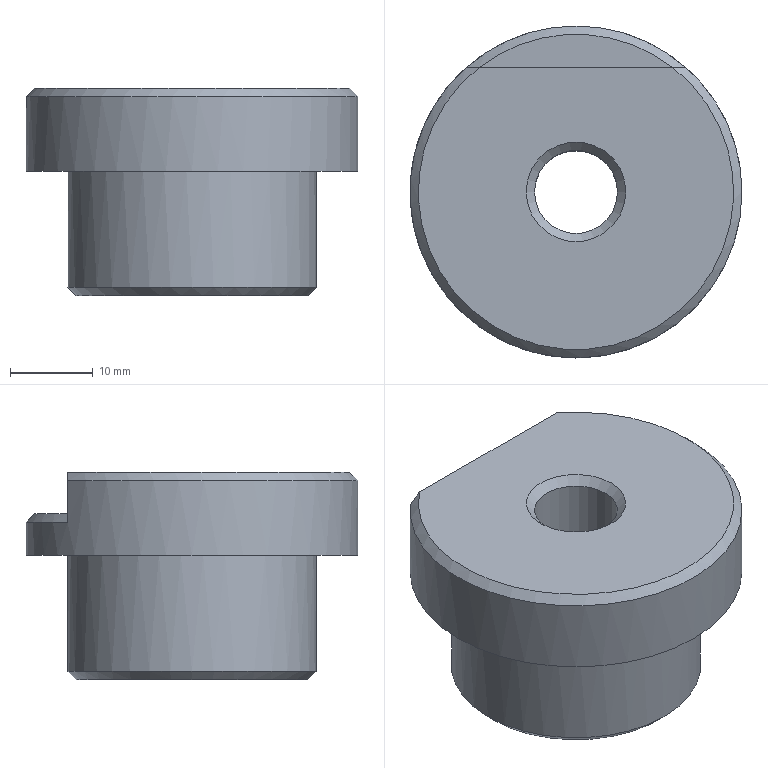Component | NX | DRILL_BUSHING_3 | 1 solid | 12 faces | box 40 x 40 x 25 mm | volume 20628 mm3 | plane 5 | cone 4 | cylinder 3 | commonest cylinder face diameters 40 x1 30 x1 10 x1
STEP:
#1=CARTESIAN_POINT('',(0.,0.,0.));
#2=DIRECTION('',(0.,0.,1.));
#3=DIRECTION('',(1.,0.,0.));
#4=AXIS2_PLACEMENT_3D('',#1,#2,#3);
#5=CARTESIAN_POINT('',(79.34,104.989,375.));
#6=VERTEX_POINT('',#5);
#7=CARTESIAN_POINT('',(59.34,104.989,375.));
#8=DIRECTION('',(0.,0.,1.));
#9=DIRECTION('',(1.,0.,0.));
#10=AXIS2_PLACEMENT_3D('',#7,#8,#9);
#11=CIRCLE('',#10,20.);
#12=CARTESIAN_POINT('',(59.34,104.989,375.));
#13=DIRECTION('',(0.,0.,1.));
#14=DIRECTION('',(1.,0.,0.));
#15=AXIS2_PLACEMENT_3D('',#12,#13,#14);
#16=CYLINDRICAL_SURFACE('',#15,20.);
#17=CARTESIAN_POINT('',(0.,0.));
#18=DIRECTION('',(1.,0.));
#19=VECTOR('',#18,1.);
#20=LINE('',#17,#19);
#21=(GEOMETRIC_REPRESENTATION_CONTEXT(2)PARAMETRIC_REPRESENTATION_CONTEXT()REPRESENTATION_CONTEXT('',''));
#22=DEFINITIONAL_REPRESENTATION('',(#20),#21);
#23=PCURVE('',#16,#22);
#24=CARTESIAN_POINT('',(59.34,104.989,375.));
#25=DIRECTION('',(0.,0.,1.));
#26=DIRECTION('',(1.,0.,0.));
#27=AXIS2_PLACEMENT_3D('',#24,#25,#26);
#28=PLANE('',#27);
#29=CARTESIAN_POINT('',(0.,0.));
#30=DIRECTION('',(1.,0.));
#31=AXIS2_PLACEMENT_2D('',#29,#30);
#32=CIRCLE('',#31,20.);
#33=(GEOMETRIC_REPRESENTATION_CONTEXT(2)PARAMETRIC_REPRESENTATION_CONTEXT()REPRESENTATION_CONTEXT('',''));
#34=DEFINITIONAL_REPRESENTATION('',(#32),#33);
#35=PCURVE('',#28,#34);
#36=SURFACE_CURVE('',#11,(#23,#35),.PCURVE_S1.);
#37=EDGE_CURVE('',#6,#6,#36,.T.);
#38=ORIENTED_EDGE('',*,*,#37,.T.);
#39=CARTESIAN_POINT('',(79.34,104.989,384.));
#40=VERTEX_POINT('',#39);
#41=CARTESIAN_POINT('',(79.34,104.989,375.));
#42=CARTESIAN_POINT('',(79.34,104.989,384.));
#43=B_SPLINE_CURVE_WITH_KNOTS('',1,(#41,#42),.UNSPECIFIED.,.F.,.F.,(2,2),(0.,9.),.PIECEWISE_BEZIER_KNOTS.);
#44=CARTESIAN_POINT('',(6.283,0.));
#45=DIRECTION('',(0.,1.));
#46=VECTOR('',#45,1.);
#47=LINE('',#44,#46);
#48=(GEOMETRIC_REPRESENTATION_CONTEXT(2)PARAMETRIC_REPRESENTATION_CONTEXT()REPRESENTATION_CONTEXT('',''));
#49=DEFINITIONAL_REPRESENTATION('',(#47),#48);
#50=PCURVE('',#16,#49);
#51=CARTESIAN_POINT('',(0.,0.));
#52=DIRECTION('',(0.,1.));
#53=VECTOR('',#52,1.);
#54=LINE('',#51,#53);
#55=(GEOMETRIC_REPRESENTATION_CONTEXT(2)PARAMETRIC_REPRESENTATION_CONTEXT()REPRESENTATION_CONTEXT('',''));
#56=DEFINITIONAL_REPRESENTATION('',(#54),#55);
#57=PCURVE('',#16,#56);
#58=SEAM_CURVE('',#43,(#50,#57),.PCURVE_S1.);
#59=EDGE_CURVE('',#6,#40,#58,.T.);
#60=ORIENTED_EDGE('',*,*,#59,.T.);
#61=CARTESIAN_POINT('',(46.111,119.989,384.));
#62=VERTEX_POINT('',#61);
#63=CARTESIAN_POINT('',(59.34,104.989,384.));
#64=DIRECTION('',(0.,0.,-1.));
#65=DIRECTION('',(1.,0.,0.));
#66=AXIS2_PLACEMENT_3D('',#63,#64,#65);
#67=CIRCLE('',#66,20.);
#68=CARTESIAN_POINT('',(12.566,9.));
#69=DIRECTION('',(-1.,0.));
#70=VECTOR('',#69,1.);
#71=LINE('',#68,#70);
#72=(GEOMETRIC_REPRESENTATION_CONTEXT(2)PARAMETRIC_REPRESENTATION_CONTEXT()REPRESENTATION_CONTEXT('',''));
#73=DEFINITIONAL_REPRESENTATION('',(#71),#72);
#74=PCURVE('',#16,#73);
#75=CARTESIAN_POINT('',(59.34,104.989,385.));
#76=DIRECTION('',(0.,0.,-1.));
#77=DIRECTION('',(-1.,0.,0.));
#78=AXIS2_PLACEMENT_3D('',#75,#76,#77);
#79=CONICAL_SURFACE('',#78,19.,0.7854);
#80=CARTESIAN_POINT('',(-3.142,1.));
#81=DIRECTION('',(1.,-0.));
#82=VECTOR('',#81,1.);
#83=LINE('',#80,#82);
#84=(GEOMETRIC_REPRESENTATION_CONTEXT(2)PARAMETRIC_REPRESENTATION_CONTEXT()REPRESENTATION_CONTEXT('',''));
#85=DEFINITIONAL_REPRESENTATION('',(#83),#84);
#86=PCURVE('',#79,#85);
#87=SURFACE_CURVE('',#67,(#74,#86),.PCURVE_S1.);
#88=EDGE_CURVE('',#40,#62,#87,.T.);
#89=ORIENTED_EDGE('',*,*,#88,.T.);
#90=CARTESIAN_POINT('',(46.111,119.989,379.));
#91=VERTEX_POINT('',#90);
#92=CARTESIAN_POINT('',(46.111,119.989,375.));
#93=DIRECTION('',(0.,0.,-1.));
#94=VECTOR('',#93,1.);
#95=LINE('',#92,#94);
#96=CARTESIAN_POINT('',(2.294,0.));
#97=DIRECTION('',(0.,-1.));
#98=VECTOR('',#97,1.);
#99=LINE('',#96,#98);
#100=(GEOMETRIC_REPRESENTATION_CONTEXT(2)PARAMETRIC_REPRESENTATION_CONTEXT()REPRESENTATION_CONTEXT('',''));
#101=DEFINITIONAL_REPRESENTATION('',(#99),#100);
#102=PCURVE('',#16,#101);
#103=CARTESIAN_POINT('',(159.34,119.989,394.));
#104=DIRECTION('',(0.,1.,0.));
#105=DIRECTION('',(0.,-0.,1.));
#106=AXIS2_PLACEMENT_3D('',#103,#104,#105);
#107=PLANE('',#106);
#108=CARTESIAN_POINT('',(-19.,-113.229));
#109=DIRECTION('',(-1.,0.));
#110=VECTOR('',#109,1.);
#111=LINE('',#108,#110);
#112=(GEOMETRIC_REPRESENTATION_CONTEXT(2)PARAMETRIC_REPRESENTATION_CONTEXT()REPRESENTATION_CONTEXT('',''));
#113=DEFINITIONAL_REPRESENTATION('',(#111),#112);
#114=PCURVE('',#107,#113);
#115=SURFACE_CURVE('',#95,(#102,#114),.PCURVE_S1.);
#116=EDGE_CURVE('',#62,#91,#115,.T.);
#117=ORIENTED_EDGE('',*,*,#116,.T.);
#118=CARTESIAN_POINT('',(72.569,119.989,379.));
#119=VERTEX_POINT('',#118);
#120=CARTESIAN_POINT('',(59.34,104.989,379.));
#121=DIRECTION('',(0.,0.,-1.));
#122=DIRECTION('',(1.,0.,0.));
#123=AXIS2_PLACEMENT_3D('',#120,#121,#122);
#124=CIRCLE('',#123,20.);
#125=CARTESIAN_POINT('',(6.283,4.));
#126=DIRECTION('',(-1.,0.));
#127=VECTOR('',#126,1.);
#128=LINE('',#125,#127);
#129=(GEOMETRIC_REPRESENTATION_CONTEXT(2)PARAMETRIC_REPRESENTATION_CONTEXT()REPRESENTATION_CONTEXT('',''));
#130=DEFINITIONAL_REPRESENTATION('',(#128),#129);
#131=PCURVE('',#16,#130);
#132=CARTESIAN_POINT('',(59.34,104.989,379.));
#133=DIRECTION('',(0.,0.,-1.));
#134=DIRECTION('',(-1.,0.,0.));
#135=AXIS2_PLACEMENT_3D('',#132,#133,#134);
#136=CONICAL_SURFACE('',#135,20.,0.7854);
#137=CARTESIAN_POINT('',(-3.142,0.));
#138=DIRECTION('',(1.,0.));
#139=VECTOR('',#138,1.);
#140=LINE('',#137,#139);
#141=(GEOMETRIC_REPRESENTATION_CONTEXT(2)PARAMETRIC_REPRESENTATION_CONTEXT()REPRESENTATION_CONTEXT('',''));
#142=DEFINITIONAL_REPRESENTATION('',(#140),#141);
#143=PCURVE('',#136,#142);
#144=SURFACE_CURVE('',#124,(#131,#143),.PCURVE_S1.);
#145=EDGE_CURVE('',#91,#119,#144,.T.);
#146=ORIENTED_EDGE('',*,*,#145,.T.);
#147=CARTESIAN_POINT('',(72.569,119.989,384.));
#148=VERTEX_POINT('',#147);
#149=CARTESIAN_POINT('',(72.569,119.989,375.));
#150=DIRECTION('',(0.,0.,1.));
#151=VECTOR('',#150,1.);
#152=LINE('',#149,#151);
#153=CARTESIAN_POINT('',(0.8481,0.));
#154=DIRECTION('',(0.,1.));
#155=VECTOR('',#154,1.);
#156=LINE('',#153,#155);
#157=(GEOMETRIC_REPRESENTATION_CONTEXT(2)PARAMETRIC_REPRESENTATION_CONTEXT()REPRESENTATION_CONTEXT('',''));
#158=DEFINITIONAL_REPRESENTATION('',(#156),#157);
#159=PCURVE('',#16,#158);
#160=CARTESIAN_POINT('',(-19.,-86.771));
#161=DIRECTION('',(1.,0.));
#162=VECTOR('',#161,1.);
#163=LINE('',#160,#162);
#164=(GEOMETRIC_REPRESENTATION_CONTEXT(2)PARAMETRIC_REPRESENTATION_CONTEXT()REPRESENTATION_CONTEXT('',''));
#165=DEFINITIONAL_REPRESENTATION('',(#163),#164);
#166=PCURVE('',#107,#165);
#167=SURFACE_CURVE('',#152,(#159,#166),.PCURVE_S1.);
#168=EDGE_CURVE('',#119,#148,#167,.T.);
#169=ORIENTED_EDGE('',*,*,#168,.T.);
#170=CARTESIAN_POINT('',(59.34,104.989,384.));
#171=DIRECTION('',(0.,0.,-1.));
#172=DIRECTION('',(1.,0.,0.));
#173=AXIS2_PLACEMENT_3D('',#170,#171,#172);
#174=CIRCLE('',#173,20.);
#175=CARTESIAN_POINT('',(6.283,9.));
#176=DIRECTION('',(-1.,0.));
#177=VECTOR('',#176,1.);
#178=LINE('',#175,#177);
#179=(GEOMETRIC_REPRESENTATION_CONTEXT(2)PARAMETRIC_REPRESENTATION_CONTEXT()REPRESENTATION_CONTEXT('',''));
#180=DEFINITIONAL_REPRESENTATION('',(#178),#179);
#181=PCURVE('',#16,#180);
#182=CARTESIAN_POINT('',(-3.142,1.));
#183=DIRECTION('',(1.,0.));
#184=VECTOR('',#183,1.);
#185=LINE('',#182,#184);
#186=(GEOMETRIC_REPRESENTATION_CONTEXT(2)PARAMETRIC_REPRESENTATION_CONTEXT()REPRESENTATION_CONTEXT('',''));
#187=DEFINITIONAL_REPRESENTATION('',(#185),#186);
#188=PCURVE('',#79,#187);
#189=SURFACE_CURVE('',#174,(#181,#188),.PCURVE_S1.);
#190=EDGE_CURVE('',#148,#40,#189,.T.);
#191=ORIENTED_EDGE('',*,*,#190,.T.);
#192=ORIENTED_EDGE('',*,*,#59,.F.);
#193=EDGE_LOOP('',(#38,#60,#89,#117,#146,#169,#191,#192));
#194=FACE_BOUND('',#193,.T.);
#195=ADVANCED_FACE('',(#194),#16,.T.);
#196=CARTESIAN_POINT('',(65.34,104.989,385.));
#197=VERTEX_POINT('',#196);
#198=CARTESIAN_POINT('',(59.34,104.989,385.));
#199=DIRECTION('',(0.,0.,-1.));
#200=DIRECTION('',(1.,0.,0.));
#201=AXIS2_PLACEMENT_3D('',#198,#199,#200);
#202=CIRCLE('',#201,6.);
#203=CARTESIAN_POINT('',(59.34,104.989,385.));
#204=DIRECTION('',(0.,0.,1.));
#205=DIRECTION('',(1.,0.,0.));
#206=AXIS2_PLACEMENT_3D('',#203,#204,#205);
#207=PLANE('',#206);
#208=CARTESIAN_POINT('',(6.,0.));
#209=CARTESIAN_POINT('',(6.,-10.392));
#210=CARTESIAN_POINT('',(-3.,-5.196));
#211=CARTESIAN_POINT('',(-12.,-0.));
#212=CARTESIAN_POINT('',(-3.,5.196));
#213=CARTESIAN_POINT('',(6.,10.392));
#214=CARTESIAN_POINT('',(6.,0.));
#215=(BOUNDED_CURVE()B_SPLINE_CURVE(2,(#208,#209,#210,#211,#212,#213,#214),.UNSPECIFIED.,.T.,.F.)B_SPLINE_CURVE_WITH_KNOTS((1,2,2,2,2,1),(-2.094,0.,2.094,4.189,6.283,8.378),.UNSPECIFIED.)CURVE()GEOMETRIC_REPRESENTATION_ITEM()RATIONAL_B_SPLINE_CURVE((1.,0.5,1.,0.5,1.,0.5,1.))REPRESENTATION_ITEM(''));
#216=(GEOMETRIC_REPRESENTATION_CONTEXT(2)PARAMETRIC_REPRESENTATION_CONTEXT()REPRESENTATION_CONTEXT('',''));
#217=DEFINITIONAL_REPRESENTATION('',(#215),#216);
#218=PCURVE('',#207,#217);
#219=CARTESIAN_POINT('',(59.34,104.989,384.));
#220=DIRECTION('',(0.,0.,1.));
#221=DIRECTION('',(1.,0.,0.));
#222=AXIS2_PLACEMENT_3D('',#219,#220,#221);
#223=CONICAL_SURFACE('',#222,5.,0.7854);
#224=CARTESIAN_POINT('',(6.283,1.));
#225=DIRECTION('',(-1.,0.));
#226=VECTOR('',#225,1.);
#227=LINE('',#224,#226);
#228=(GEOMETRIC_REPRESENTATION_CONTEXT(2)PARAMETRIC_REPRESENTATION_CONTEXT()REPRESENTATION_CONTEXT('',''));
#229=DEFINITIONAL_REPRESENTATION('',(#227),#228);
#230=PCURVE('',#223,#229);
#231=SURFACE_CURVE('',#202,(#218,#230),.PCURVE_S1.);
#232=EDGE_CURVE('',#197,#197,#231,.T.);
#233=ORIENTED_EDGE('',*,*,#232,.T.);
#234=EDGE_LOOP('',(#233));
#235=FACE_BOUND('',#234,.T.);
#236=CARTESIAN_POINT('',(71.002,119.989,385.));
#237=VERTEX_POINT('',#236);
#238=CARTESIAN_POINT('',(47.678,119.989,385.));
#239=VERTEX_POINT('',#238);
#240=CARTESIAN_POINT('',(59.34,119.989,385.));
#241=DIRECTION('',(-1.,0.,0.));
#242=VECTOR('',#241,1.);
#243=LINE('',#240,#242);
#244=CARTESIAN_POINT('',(0.,15.));
#245=DIRECTION('',(-1.,0.));
#246=VECTOR('',#245,1.);
#247=LINE('',#244,#246);
#248=(GEOMETRIC_REPRESENTATION_CONTEXT(2)PARAMETRIC_REPRESENTATION_CONTEXT()REPRESENTATION_CONTEXT('',''));
#249=DEFINITIONAL_REPRESENTATION('',(#247),#248);
#250=PCURVE('',#207,#249);
#251=CARTESIAN_POINT('',(-9.,-100.));
#252=DIRECTION('',(0.,-1.));
#253=VECTOR('',#252,1.);
#254=LINE('',#251,#253);
#255=(GEOMETRIC_REPRESENTATION_CONTEXT(2)PARAMETRIC_REPRESENTATION_CONTEXT()REPRESENTATION_CONTEXT('',''));
#256=DEFINITIONAL_REPRESENTATION('',(#254),#255);
#257=PCURVE('',#107,#256);
#258=SURFACE_CURVE('',#243,(#250,#257),.PCURVE_S1.);
#259=EDGE_CURVE('',#237,#239,#258,.T.);
#260=ORIENTED_EDGE('',*,*,#259,.T.);
#261=CARTESIAN_POINT('',(59.34,104.989,385.));
#262=DIRECTION('',(0.,0.,1.));
#263=DIRECTION('',(1.,0.,0.));
#264=AXIS2_PLACEMENT_3D('',#261,#262,#263);
#265=CIRCLE('',#264,19.);
#266=CARTESIAN_POINT('',(0.,0.));
#267=DIRECTION('',(1.,0.));
#268=AXIS2_PLACEMENT_2D('',#266,#267);
#269=CIRCLE('',#268,19.);
#270=(GEOMETRIC_REPRESENTATION_CONTEXT(2)PARAMETRIC_REPRESENTATION_CONTEXT()REPRESENTATION_CONTEXT('',''));
#271=DEFINITIONAL_REPRESENTATION('',(#269),#270);
#272=PCURVE('',#207,#271);
#273=CARTESIAN_POINT('',(9.425,0.));
#274=DIRECTION('',(-1.,-0.));
#275=VECTOR('',#274,1.);
#276=LINE('',#273,#275);
#277=(GEOMETRIC_REPRESENTATION_CONTEXT(2)PARAMETRIC_REPRESENTATION_CONTEXT()REPRESENTATION_CONTEXT('',''));
#278=DEFINITIONAL_REPRESENTATION('',(#276),#277);
#279=PCURVE('',#79,#278);
#280=SURFACE_CURVE('',#265,(#272,#279),.PCURVE_S1.);
#281=EDGE_CURVE('',#239,#237,#280,.T.);
#282=ORIENTED_EDGE('',*,*,#281,.T.);
#283=EDGE_LOOP('',(#260,#282));
#284=FACE_BOUND('',#283,.T.);
#285=ADVANCED_FACE('',(#235,#284),#207,.T.);
#286=CARTESIAN_POINT('',(74.34,104.989,375.));
#287=VERTEX_POINT('',#286);
#288=CARTESIAN_POINT('',(59.34,104.989,375.));
#289=DIRECTION('',(0.,0.,-1.));
#290=DIRECTION('',(1.,0.,0.));
#291=AXIS2_PLACEMENT_3D('',#288,#289,#290);
#292=CIRCLE('',#291,15.);
#293=CARTESIAN_POINT('',(15.,0.));
#294=CARTESIAN_POINT('',(15.,-25.981));
#295=CARTESIAN_POINT('',(-7.5,-12.99));
#296=CARTESIAN_POINT('',(-30.,-0.));
#297=CARTESIAN_POINT('',(-7.5,12.99));
#298=CARTESIAN_POINT('',(15.,25.981));
#299=CARTESIAN_POINT('',(15.,0.));
#300=(BOUNDED_CURVE()B_SPLINE_CURVE(2,(#293,#294,#295,#296,#297,#298,#299),.UNSPECIFIED.,.T.,.F.)B_SPLINE_CURVE_WITH_KNOTS((1,2,2,2,2,1),(-2.094,0.,2.094,4.189,6.283,8.378),.UNSPECIFIED.)CURVE()GEOMETRIC_REPRESENTATION_ITEM()RATIONAL_B_SPLINE_CURVE((1.,0.5,1.,0.5,1.,0.5,1.))REPRESENTATION_ITEM(''));
#301=(GEOMETRIC_REPRESENTATION_CONTEXT(2)PARAMETRIC_REPRESENTATION_CONTEXT()REPRESENTATION_CONTEXT('',''));
#302=DEFINITIONAL_REPRESENTATION('',(#300),#301);
#303=PCURVE('',#28,#302);
#304=CARTESIAN_POINT('',(59.34,104.989,360.));
#305=DIRECTION('',(0.,0.,1.));
#306=DIRECTION('',(1.,0.,0.));
#307=AXIS2_PLACEMENT_3D('',#304,#305,#306);
#308=CYLINDRICAL_SURFACE('',#307,15.);
#309=CARTESIAN_POINT('',(6.283,15.));
#310=DIRECTION('',(-1.,0.));
#311=VECTOR('',#310,1.);
#312=LINE('',#309,#311);
#313=(GEOMETRIC_REPRESENTATION_CONTEXT(2)PARAMETRIC_REPRESENTATION_CONTEXT()REPRESENTATION_CONTEXT('',''));
#314=DEFINITIONAL_REPRESENTATION('',(#312),#313);
#315=PCURVE('',#308,#314);
#316=SURFACE_CURVE('',#292,(#303,#315),.PCURVE_S1.);
#317=EDGE_CURVE('',#287,#287,#316,.T.);
#318=ORIENTED_EDGE('',*,*,#317,.F.);
#319=EDGE_LOOP('',(#318));
#320=FACE_BOUND('',#319,.T.);
#321=ORIENTED_EDGE('',*,*,#37,.F.);
#322=EDGE_LOOP('',(#321));
#323=FACE_BOUND('',#322,.T.);
#324=ADVANCED_FACE('',(#320,#323),#28,.F.);
#325=CARTESIAN_POINT('',(44.34,104.989,361.));
#326=VERTEX_POINT('',#325);
#327=CARTESIAN_POINT('',(74.34,104.989,361.));
#328=VERTEX_POINT('',#327);
#329=CARTESIAN_POINT('',(59.34,104.989,361.));
#330=DIRECTION('',(0.,0.,1.));
#331=DIRECTION('',(-1.,0.,0.));
#332=AXIS2_PLACEMENT_3D('',#329,#330,#331);
#333=CIRCLE('',#332,15.);
#334=CARTESIAN_POINT('',(3.142,1.));
#335=DIRECTION('',(1.,0.));
#336=VECTOR('',#335,1.);
#337=LINE('',#334,#336);
#338=(GEOMETRIC_REPRESENTATION_CONTEXT(2)PARAMETRIC_REPRESENTATION_CONTEXT()REPRESENTATION_CONTEXT('',''));
#339=DEFINITIONAL_REPRESENTATION('',(#337),#338);
#340=PCURVE('',#308,#339);
#341=CARTESIAN_POINT('',(59.34,104.989,360.));
#342=DIRECTION('',(0.,0.,1.));
#343=DIRECTION('',(1.,0.,0.));
#344=AXIS2_PLACEMENT_3D('',#341,#342,#343);
#345=CONICAL_SURFACE('',#344,14.,0.7854);
#346=CARTESIAN_POINT('',(3.142,1.));
#347=DIRECTION('',(1.,0.));
#348=VECTOR('',#347,1.);
#349=LINE('',#346,#348);
#350=(GEOMETRIC_REPRESENTATION_CONTEXT(2)PARAMETRIC_REPRESENTATION_CONTEXT()REPRESENTATION_CONTEXT('',''));
#351=DEFINITIONAL_REPRESENTATION('',(#349),#350);
#352=PCURVE('',#345,#351);
#353=SURFACE_CURVE('',#333,(#340,#352),.PCURVE_S1.);
#354=EDGE_CURVE('',#326,#328,#353,.T.);
#355=ORIENTED_EDGE('',*,*,#354,.T.);
#356=CARTESIAN_POINT('',(74.34,104.989,361.));
#357=CARTESIAN_POINT('',(74.34,104.989,375.));
#358=B_SPLINE_CURVE_WITH_KNOTS('',1,(#356,#357),.UNSPECIFIED.,.F.,.F.,(2,2),(1.,15.),.PIECEWISE_BEZIER_KNOTS.);
#359=CARTESIAN_POINT('',(6.283,0.));
#360=DIRECTION('',(0.,1.));
#361=VECTOR('',#360,1.);
#362=LINE('',#359,#361);
#363=(GEOMETRIC_REPRESENTATION_CONTEXT(2)PARAMETRIC_REPRESENTATION_CONTEXT()REPRESENTATION_CONTEXT('',''));
#364=DEFINITIONAL_REPRESENTATION('',(#362),#363);
#365=PCURVE('',#308,#364);
#366=CARTESIAN_POINT('',(0.,0.));
#367=DIRECTION('',(0.,1.));
#368=VECTOR('',#367,1.);
#369=LINE('',#366,#368);
#370=(GEOMETRIC_REPRESENTATION_CONTEXT(2)PARAMETRIC_REPRESENTATION_CONTEXT()REPRESENTATION_CONTEXT('',''));
#371=DEFINITIONAL_REPRESENTATION('',(#369),#370);
#372=PCURVE('',#308,#371);
#373=SEAM_CURVE('',#358,(#365,#372),.PCURVE_S1.);
#374=EDGE_CURVE('',#328,#287,#373,.T.);
#375=ORIENTED_EDGE('',*,*,#374,.T.);
#376=ORIENTED_EDGE('',*,*,#317,.T.);
#377=ORIENTED_EDGE('',*,*,#374,.F.);
#378=CARTESIAN_POINT('',(59.34,104.989,361.));
#379=DIRECTION('',(0.,0.,1.));
#380=DIRECTION('',(-1.,0.,0.));
#381=AXIS2_PLACEMENT_3D('',#378,#379,#380);
#382=CIRCLE('',#381,15.);
#383=CARTESIAN_POINT('',(-3.142,1.));
#384=DIRECTION('',(1.,0.));
#385=VECTOR('',#384,1.);
#386=LINE('',#383,#385);
#387=(GEOMETRIC_REPRESENTATION_CONTEXT(2)PARAMETRIC_REPRESENTATION_CONTEXT()REPRESENTATION_CONTEXT('',''));
#388=DEFINITIONAL_REPRESENTATION('',(#386),#387);
#389=PCURVE('',#308,#388);
#390=CARTESIAN_POINT('',(3.142,1.));
#391=DIRECTION('',(1.,-0.));
#392=VECTOR('',#391,1.);
#393=LINE('',#390,#392);
#394=(GEOMETRIC_REPRESENTATION_CONTEXT(2)PARAMETRIC_REPRESENTATION_CONTEXT()REPRESENTATION_CONTEXT('',''));
#395=DEFINITIONAL_REPRESENTATION('',(#393),#394);
#396=PCURVE('',#345,#395);
#397=SURFACE_CURVE('',#382,(#389,#396),.PCURVE_S1.);
#398=EDGE_CURVE('',#328,#326,#397,.T.);
#399=ORIENTED_EDGE('',*,*,#398,.T.);
#400=EDGE_LOOP('',(#355,#375,#376,#377,#399));
#401=FACE_BOUND('',#400,.T.);
#402=ADVANCED_FACE('',(#401),#308,.T.);
#403=CARTESIAN_POINT('',(45.34,104.989,360.));
#404=VERTEX_POINT('',#403);
#405=CARTESIAN_POINT('',(59.34,104.989,360.));
#406=DIRECTION('',(0.,0.,-1.));
#407=DIRECTION('',(-1.,0.,0.));
#408=AXIS2_PLACEMENT_3D('',#405,#406,#407);
#409=CIRCLE('',#408,14.);
#410=CARTESIAN_POINT('',(59.34,104.989,360.));
#411=DIRECTION('',(0.,0.,-1.));
#412=DIRECTION('',(-1.,0.,0.));
#413=AXIS2_PLACEMENT_3D('',#410,#411,#412);
#414=PLANE('',#413);
#415=CARTESIAN_POINT('',(0.,0.));
#416=DIRECTION('',(1.,0.));
#417=AXIS2_PLACEMENT_2D('',#415,#416);
#418=CIRCLE('',#417,14.);
#419=(GEOMETRIC_REPRESENTATION_CONTEXT(2)PARAMETRIC_REPRESENTATION_CONTEXT()REPRESENTATION_CONTEXT('',''));
#420=DEFINITIONAL_REPRESENTATION('',(#418),#419);
#421=PCURVE('',#414,#420);
#422=CARTESIAN_POINT('',(9.425,0.));
#423=DIRECTION('',(-1.,0.));
#424=VECTOR('',#423,1.);
#425=LINE('',#422,#424);
#426=(GEOMETRIC_REPRESENTATION_CONTEXT(2)PARAMETRIC_REPRESENTATION_CONTEXT()REPRESENTATION_CONTEXT('',''));
#427=DEFINITIONAL_REPRESENTATION('',(#425),#426);
#428=PCURVE('',#345,#427);
#429=SURFACE_CURVE('',#409,(#421,#428),.PCURVE_S1.);
#430=EDGE_CURVE('',#404,#404,#429,.T.);
#431=ORIENTED_EDGE('',*,*,#430,.T.);
#432=EDGE_LOOP('',(#431));
#433=FACE_BOUND('',#432,.T.);
#434=CARTESIAN_POINT('',(54.34,104.989,360.));
#435=VERTEX_POINT('',#434);
#436=CARTESIAN_POINT('',(64.34,104.989,360.));
#437=VERTEX_POINT('',#436);
#438=CARTESIAN_POINT('',(59.34,104.989,360.));
#439=DIRECTION('',(0.,0.,-1.));
#440=DIRECTION('',(-1.,0.,0.));
#441=AXIS2_PLACEMENT_3D('',#438,#439,#440);
#442=CIRCLE('',#441,5.);
#443=CARTESIAN_POINT('',(0.,0.));
#444=DIRECTION('',(1.,0.));
#445=AXIS2_PLACEMENT_2D('',#443,#444);
#446=CIRCLE('',#445,5.);
#447=(GEOMETRIC_REPRESENTATION_CONTEXT(2)PARAMETRIC_REPRESENTATION_CONTEXT()REPRESENTATION_CONTEXT('',''));
#448=DEFINITIONAL_REPRESENTATION('',(#446),#447);
#449=PCURVE('',#414,#448);
#450=CARTESIAN_POINT('',(59.34,104.989,285.));
#451=DIRECTION('',(0.,0.,1.));
#452=DIRECTION('',(1.,0.,0.));
#453=AXIS2_PLACEMENT_3D('',#450,#451,#452);
#454=CYLINDRICAL_SURFACE('',#453,5.);
#455=CARTESIAN_POINT('',(3.142,75.));
#456=DIRECTION('',(-1.,0.));
#457=VECTOR('',#456,1.);
#458=LINE('',#455,#457);
#459=(GEOMETRIC_REPRESENTATION_CONTEXT(2)PARAMETRIC_REPRESENTATION_CONTEXT()REPRESENTATION_CONTEXT('',''));
#460=DEFINITIONAL_REPRESENTATION('',(#458),#459);
#461=PCURVE('',#454,#460);
#462=SURFACE_CURVE('',#442,(#449,#461),.PCURVE_S1.);
#463=EDGE_CURVE('',#435,#437,#462,.T.);
#464=ORIENTED_EDGE('',*,*,#463,.F.);
#465=CARTESIAN_POINT('',(59.34,104.989,360.));
#466=DIRECTION('',(0.,0.,-1.));
#467=DIRECTION('',(-1.,0.,0.));
#468=AXIS2_PLACEMENT_3D('',#465,#466,#467);
#469=CIRCLE('',#468,5.);
#470=CARTESIAN_POINT('',(0.,0.));
#471=DIRECTION('',(1.,0.));
#472=AXIS2_PLACEMENT_2D('',#470,#471);
#473=CIRCLE('',#472,5.);
#474=(GEOMETRIC_REPRESENTATION_CONTEXT(2)PARAMETRIC_REPRESENTATION_CONTEXT()REPRESENTATION_CONTEXT('',''));
#475=DEFINITIONAL_REPRESENTATION('',(#473),#474);
#476=PCURVE('',#414,#475);
#477=CARTESIAN_POINT('',(9.425,75.));
#478=DIRECTION('',(-1.,0.));
#479=VECTOR('',#478,1.);
#480=LINE('',#477,#479);
#481=(GEOMETRIC_REPRESENTATION_CONTEXT(2)PARAMETRIC_REPRESENTATION_CONTEXT()REPRESENTATION_CONTEXT('',''));
#482=DEFINITIONAL_REPRESENTATION('',(#480),#481);
#483=PCURVE('',#454,#482);
#484=SURFACE_CURVE('',#469,(#476,#483),.PCURVE_S1.);
#485=EDGE_CURVE('',#437,#435,#484,.T.);
#486=ORIENTED_EDGE('',*,*,#485,.F.);
#487=EDGE_LOOP('',(#464,#486));
#488=FACE_BOUND('',#487,.T.);
#489=ADVANCED_FACE('',(#433,#488),#414,.T.);
#490=CARTESIAN_POINT('',(64.34,104.989,384.));
#491=VERTEX_POINT('',#490);
#492=CARTESIAN_POINT('',(59.34,104.989,384.));
#493=DIRECTION('',(0.,0.,1.));
#494=DIRECTION('',(1.,0.,0.));
#495=AXIS2_PLACEMENT_3D('',#492,#493,#494);
#496=CIRCLE('',#495,5.);
#497=CARTESIAN_POINT('',(0.,99.));
#498=DIRECTION('',(1.,0.));
#499=VECTOR('',#498,1.);
#500=LINE('',#497,#499);
#501=(GEOMETRIC_REPRESENTATION_CONTEXT(2)PARAMETRIC_REPRESENTATION_CONTEXT()REPRESENTATION_CONTEXT('',''));
#502=DEFINITIONAL_REPRESENTATION('',(#500),#501);
#503=PCURVE('',#454,#502);
#504=CARTESIAN_POINT('',(0.,0.));
#505=DIRECTION('',(1.,0.));
#506=VECTOR('',#505,1.);
#507=LINE('',#504,#506);
#508=(GEOMETRIC_REPRESENTATION_CONTEXT(2)PARAMETRIC_REPRESENTATION_CONTEXT()REPRESENTATION_CONTEXT('',''));
#509=DEFINITIONAL_REPRESENTATION('',(#507),#508);
#510=PCURVE('',#223,#509);
#511=SURFACE_CURVE('',#496,(#503,#510),.PCURVE_S1.);
#512=EDGE_CURVE('',#491,#491,#511,.T.);
#513=ORIENTED_EDGE('',*,*,#512,.F.);
#514=CARTESIAN_POINT('',(64.34,104.989,360.));
#515=CARTESIAN_POINT('',(64.34,104.989,384.));
#516=B_SPLINE_CURVE_WITH_KNOTS('',1,(#514,#515),.UNSPECIFIED.,.F.,.F.,(2,2),(75.,99.),.PIECEWISE_BEZIER_KNOTS.);
#517=CARTESIAN_POINT('',(0.,0.));
#518=DIRECTION('',(0.,1.));
#519=VECTOR('',#518,1.);
#520=LINE('',#517,#519);
#521=(GEOMETRIC_REPRESENTATION_CONTEXT(2)PARAMETRIC_REPRESENTATION_CONTEXT()REPRESENTATION_CONTEXT('',''));
#522=DEFINITIONAL_REPRESENTATION('',(#520),#521);
#523=PCURVE('',#454,#522);
#524=CARTESIAN_POINT('',(6.283,0.));
#525=DIRECTION('',(0.,1.));
#526=VECTOR('',#525,1.);
#527=LINE('',#524,#526);
#528=(GEOMETRIC_REPRESENTATION_CONTEXT(2)PARAMETRIC_REPRESENTATION_CONTEXT()REPRESENTATION_CONTEXT('',''));
#529=DEFINITIONAL_REPRESENTATION('',(#527),#528);
#530=PCURVE('',#454,#529);
#531=SEAM_CURVE('',#516,(#523,#530),.PCURVE_S1.);
#532=EDGE_CURVE('',#437,#491,#531,.T.);
#533=ORIENTED_EDGE('',*,*,#532,.F.);
#534=ORIENTED_EDGE('',*,*,#463,.F.);
#535=ORIENTED_EDGE('',*,*,#485,.F.);
#536=ORIENTED_EDGE('',*,*,#532,.T.);
#537=EDGE_LOOP('',(#513,#533,#534,#535,#536));
#538=FACE_BOUND('',#537,.F.);
#539=ADVANCED_FACE('',(#538),#454,.F.);
#540=ORIENTED_EDGE('',*,*,#259,.F.);
#541=CARTESIAN_POINT('',(71.002,119.989,385.));
#542=CARTESIAN_POINT('',(71.53,119.989,384.676));
#543=CARTESIAN_POINT('',(72.052,119.989,384.342));
#544=CARTESIAN_POINT('',(72.569,119.989,384.));
#545=B_SPLINE_CURVE_WITH_KNOTS('',3,(#541,#542,#543,#544),.UNSPECIFIED.,.F.,.F.,(4,4),(0.,1.),.PIECEWISE_BEZIER_KNOTS.);
#546=CARTESIAN_POINT('',(-9.,-88.338));
#547=CARTESIAN_POINT('',(-9.324,-87.81));
#548=CARTESIAN_POINT('',(-9.658,-87.288));
#549=CARTESIAN_POINT('',(-10.,-86.771));
#550=B_SPLINE_CURVE_WITH_KNOTS('',3,(#546,#547,#548,#549),.UNSPECIFIED.,.F.,.F.,(4,4),(0.,1.),.PIECEWISE_BEZIER_KNOTS.);
#551=(GEOMETRIC_REPRESENTATION_CONTEXT(2)PARAMETRIC_REPRESENTATION_CONTEXT()REPRESENTATION_CONTEXT('',''));
#552=DEFINITIONAL_REPRESENTATION('',(#550),#551);
#553=PCURVE('',#107,#552);
#554=CARTESIAN_POINT('',(2.232,0.));
#555=CARTESIAN_POINT('',(2.294,1.));
#556=B_SPLINE_CURVE_WITH_KNOTS('',1,(#554,#555),.UNSPECIFIED.,.F.,.F.,(2,2),(0.,1.),.PIECEWISE_BEZIER_KNOTS.);
#557=(GEOMETRIC_REPRESENTATION_CONTEXT(2)PARAMETRIC_REPRESENTATION_CONTEXT()REPRESENTATION_CONTEXT('',''));
#558=DEFINITIONAL_REPRESENTATION('',(#556),#557);
#559=PCURVE('',#79,#558);
#560=SURFACE_CURVE('',#545,(#553,#559),.PCURVE_S1.);
#561=EDGE_CURVE('',#237,#148,#560,.T.);
#562=ORIENTED_EDGE('',*,*,#561,.T.);
#563=ORIENTED_EDGE('',*,*,#168,.F.);
#564=CARTESIAN_POINT('',(71.002,119.989,380.));
#565=VERTEX_POINT('',#564);
#566=CARTESIAN_POINT('',(72.569,119.989,379.));
#567=CARTESIAN_POINT('',(72.052,119.989,379.342));
#568=CARTESIAN_POINT('',(71.53,119.989,379.676));
#569=CARTESIAN_POINT('',(71.002,119.989,380.));
#570=B_SPLINE_CURVE_WITH_KNOTS('',3,(#566,#567,#568,#569),.UNSPECIFIED.,.F.,.F.,(4,4),(0.,1.),.PIECEWISE_BEZIER_KNOTS.);
#571=CARTESIAN_POINT('',(-15.,-86.771));
#572=CARTESIAN_POINT('',(-14.658,-87.288));
#573=CARTESIAN_POINT('',(-14.324,-87.81));
#574=CARTESIAN_POINT('',(-14.,-88.338));
#575=B_SPLINE_CURVE_WITH_KNOTS('',3,(#571,#572,#573,#574),.UNSPECIFIED.,.F.,.F.,(4,4),(0.,1.),.PIECEWISE_BEZIER_KNOTS.);
#576=(GEOMETRIC_REPRESENTATION_CONTEXT(2)PARAMETRIC_REPRESENTATION_CONTEXT()REPRESENTATION_CONTEXT('',''));
#577=DEFINITIONAL_REPRESENTATION('',(#575),#576);
#578=PCURVE('',#107,#577);
#579=CARTESIAN_POINT('',(2.294,0.));
#580=CARTESIAN_POINT('',(2.232,-1.));
#581=B_SPLINE_CURVE_WITH_KNOTS('',1,(#579,#580),.UNSPECIFIED.,.F.,.F.,(2,2),(0.,1.),.PIECEWISE_BEZIER_KNOTS.);
#582=(GEOMETRIC_REPRESENTATION_CONTEXT(2)PARAMETRIC_REPRESENTATION_CONTEXT()REPRESENTATION_CONTEXT('',''));
#583=DEFINITIONAL_REPRESENTATION('',(#581),#582);
#584=PCURVE('',#136,#583);
#585=SURFACE_CURVE('',#570,(#578,#584),.PCURVE_S1.);
#586=EDGE_CURVE('',#119,#565,#585,.T.);
#587=ORIENTED_EDGE('',*,*,#586,.T.);
#588=CARTESIAN_POINT('',(47.678,119.989,380.));
#589=VERTEX_POINT('',#588);
#590=CARTESIAN_POINT('',(159.34,119.989,380.));
#591=DIRECTION('',(1.,0.,0.));
#592=VECTOR('',#591,1.);
#593=LINE('',#590,#592);
#594=CARTESIAN_POINT('',(-14.,0.));
#595=DIRECTION('',(0.,1.));
#596=VECTOR('',#595,1.);
#597=LINE('',#594,#596);
#598=(GEOMETRIC_REPRESENTATION_CONTEXT(2)PARAMETRIC_REPRESENTATION_CONTEXT()REPRESENTATION_CONTEXT('',''));
#599=DEFINITIONAL_REPRESENTATION('',(#597),#598);
#600=PCURVE('',#107,#599);
#601=CARTESIAN_POINT('',(159.34,119.989,380.));
#602=DIRECTION('',(0.,-0.,1.));
#603=DIRECTION('',(0.,-1.,-0.));
#604=AXIS2_PLACEMENT_3D('',#601,#602,#603);
#605=PLANE('',#604);
#606=CARTESIAN_POINT('',(0.,0.));
#607=DIRECTION('',(0.,1.));
#608=VECTOR('',#607,1.);
#609=LINE('',#606,#608);
#610=(GEOMETRIC_REPRESENTATION_CONTEXT(2)PARAMETRIC_REPRESENTATION_CONTEXT()REPRESENTATION_CONTEXT('',''));
#611=DEFINITIONAL_REPRESENTATION('',(#609),#610);
#612=PCURVE('',#605,#611);
#613=SURFACE_CURVE('',#593,(#600,#612),.PCURVE_S1.);
#614=EDGE_CURVE('',#589,#565,#613,.T.);
#615=ORIENTED_EDGE('',*,*,#614,.F.);
#616=CARTESIAN_POINT('',(47.678,119.989,380.));
#617=CARTESIAN_POINT('',(47.15,119.989,379.676));
#618=CARTESIAN_POINT('',(46.628,119.989,379.342));
#619=CARTESIAN_POINT('',(46.111,119.989,379.));
#620=B_SPLINE_CURVE_WITH_KNOTS('',3,(#616,#617,#618,#619),.UNSPECIFIED.,.F.,.F.,(4,4),(0.,1.),.PIECEWISE_BEZIER_KNOTS.);
#621=CARTESIAN_POINT('',(-14.,-111.662));
#622=CARTESIAN_POINT('',(-14.324,-112.19));
#623=CARTESIAN_POINT('',(-14.658,-112.712));
#624=CARTESIAN_POINT('',(-15.,-113.229));
#625=B_SPLINE_CURVE_WITH_KNOTS('',3,(#621,#622,#623,#624),.UNSPECIFIED.,.F.,.F.,(4,4),(0.,1.),.PIECEWISE_BEZIER_KNOTS.);
#626=(GEOMETRIC_REPRESENTATION_CONTEXT(2)PARAMETRIC_REPRESENTATION_CONTEXT()REPRESENTATION_CONTEXT('',''));
#627=DEFINITIONAL_REPRESENTATION('',(#625),#626);
#628=PCURVE('',#107,#627);
#629=CARTESIAN_POINT('',(0.91,-1.));
#630=CARTESIAN_POINT('',(0.8481,-0.));
#631=B_SPLINE_CURVE_WITH_KNOTS('',1,(#629,#630),.UNSPECIFIED.,.F.,.F.,(2,2),(0.,1.),.PIECEWISE_BEZIER_KNOTS.);
#632=(GEOMETRIC_REPRESENTATION_CONTEXT(2)PARAMETRIC_REPRESENTATION_CONTEXT()REPRESENTATION_CONTEXT('',''));
#633=DEFINITIONAL_REPRESENTATION('',(#631),#632);
#634=PCURVE('',#136,#633);
#635=SURFACE_CURVE('',#620,(#628,#634),.PCURVE_S1.);
#636=EDGE_CURVE('',#589,#91,#635,.T.);
#637=ORIENTED_EDGE('',*,*,#636,.T.);
#638=ORIENTED_EDGE('',*,*,#116,.F.);
#639=CARTESIAN_POINT('',(46.111,119.989,384.));
#640=CARTESIAN_POINT('',(46.628,119.989,384.342));
#641=CARTESIAN_POINT('',(47.15,119.989,384.676));
#642=CARTESIAN_POINT('',(47.678,119.989,385.));
#643=B_SPLINE_CURVE_WITH_KNOTS('',3,(#639,#640,#641,#642),.UNSPECIFIED.,.F.,.F.,(4,4),(0.,1.),.PIECEWISE_BEZIER_KNOTS.);
#644=CARTESIAN_POINT('',(-10.,-113.229));
#645=CARTESIAN_POINT('',(-9.658,-112.712));
#646=CARTESIAN_POINT('',(-9.324,-112.19));
#647=CARTESIAN_POINT('',(-9.,-111.662));
#648=B_SPLINE_CURVE_WITH_KNOTS('',3,(#644,#645,#646,#647),.UNSPECIFIED.,.F.,.F.,(4,4),(0.,1.),.PIECEWISE_BEZIER_KNOTS.);
#649=(GEOMETRIC_REPRESENTATION_CONTEXT(2)PARAMETRIC_REPRESENTATION_CONTEXT()REPRESENTATION_CONTEXT('',''));
#650=DEFINITIONAL_REPRESENTATION('',(#648),#649);
#651=PCURVE('',#107,#650);
#652=CARTESIAN_POINT('',(7.131,1.));
#653=CARTESIAN_POINT('',(7.193,0.));
#654=B_SPLINE_CURVE_WITH_KNOTS('',1,(#652,#653),.UNSPECIFIED.,.F.,.F.,(2,2),(0.,1.),.PIECEWISE_BEZIER_KNOTS.);
#655=(GEOMETRIC_REPRESENTATION_CONTEXT(2)PARAMETRIC_REPRESENTATION_CONTEXT()REPRESENTATION_CONTEXT('',''));
#656=DEFINITIONAL_REPRESENTATION('',(#654),#655);
#657=PCURVE('',#79,#656);
#658=SURFACE_CURVE('',#643,(#651,#657),.PCURVE_S1.);
#659=EDGE_CURVE('',#62,#239,#658,.T.);
#660=ORIENTED_EDGE('',*,*,#659,.T.);
#661=EDGE_LOOP('',(#540,#562,#563,#587,#615,#637,#638,#660));
#662=FACE_BOUND('',#661,.T.);
#663=ADVANCED_FACE('',(#662),#107,.T.);
#664=ORIENTED_EDGE('',*,*,#614,.T.);
#665=CARTESIAN_POINT('',(59.34,104.989,380.));
#666=DIRECTION('',(0.,-0.,1.));
#667=DIRECTION('',(0.,-1.,-0.));
#668=AXIS2_PLACEMENT_3D('',#665,#666,#667);
#669=CIRCLE('',#668,19.);
#670=CARTESIAN_POINT('',(15.,-100.));
#671=DIRECTION('',(1.,0.));
#672=AXIS2_PLACEMENT_2D('',#670,#671);
#673=CIRCLE('',#672,19.);
#674=(GEOMETRIC_REPRESENTATION_CONTEXT(2)PARAMETRIC_REPRESENTATION_CONTEXT()REPRESENTATION_CONTEXT('',''));
#675=DEFINITIONAL_REPRESENTATION('',(#673),#674);
#676=PCURVE('',#605,#675);
#677=CARTESIAN_POINT('',(4.712,-1.));
#678=DIRECTION('',(-1.,-0.));
#679=VECTOR('',#678,1.);
#680=LINE('',#677,#679);
#681=(GEOMETRIC_REPRESENTATION_CONTEXT(2)PARAMETRIC_REPRESENTATION_CONTEXT()REPRESENTATION_CONTEXT('',''));
#682=DEFINITIONAL_REPRESENTATION('',(#680),#681);
#683=PCURVE('',#136,#682);
#684=SURFACE_CURVE('',#669,(#676,#683),.PCURVE_S1.);
#685=EDGE_CURVE('',#565,#589,#684,.T.);
#686=ORIENTED_EDGE('',*,*,#685,.T.);
#687=EDGE_LOOP('',(#664,#686));
#688=FACE_BOUND('',#687,.T.);
#689=ADVANCED_FACE('',(#688),#605,.T.);
#690=ORIENTED_EDGE('',*,*,#659,.F.);
#691=ORIENTED_EDGE('',*,*,#88,.F.);
#692=ORIENTED_EDGE('',*,*,#190,.F.);
#693=ORIENTED_EDGE('',*,*,#561,.F.);
#694=ORIENTED_EDGE('',*,*,#281,.F.);
#695=EDGE_LOOP('',(#690,#691,#692,#693,#694));
#696=FACE_BOUND('',#695,.T.);
#697=ADVANCED_FACE('',(#696),#79,.T.);
#698=ORIENTED_EDGE('',*,*,#232,.T.);
#699=CARTESIAN_POINT('',(64.34,104.989,384.));
#700=CARTESIAN_POINT('',(65.34,104.989,385.));
#701=B_SPLINE_CURVE_WITH_KNOTS('',1,(#699,#700),.UNSPECIFIED.,.F.,.F.,(2,2),(0.,1.414),.PIECEWISE_BEZIER_KNOTS.);
#702=CARTESIAN_POINT('',(0.,0.));
#703=DIRECTION('',(0.,1.));
#704=VECTOR('',#703,1.);
#705=LINE('',#702,#704);
#706=(GEOMETRIC_REPRESENTATION_CONTEXT(2)PARAMETRIC_REPRESENTATION_CONTEXT()REPRESENTATION_CONTEXT('',''));
#707=DEFINITIONAL_REPRESENTATION('',(#705),#706);
#708=PCURVE('',#223,#707);
#709=CARTESIAN_POINT('',(6.283,0.));
#710=DIRECTION('',(0.,1.));
#711=VECTOR('',#710,1.);
#712=LINE('',#709,#711);
#713=(GEOMETRIC_REPRESENTATION_CONTEXT(2)PARAMETRIC_REPRESENTATION_CONTEXT()REPRESENTATION_CONTEXT('',''));
#714=DEFINITIONAL_REPRESENTATION('',(#712),#713);
#715=PCURVE('',#223,#714);
#716=SEAM_CURVE('',#701,(#708,#715),.PCURVE_S1.);
#717=EDGE_CURVE('',#491,#197,#716,.T.);
#718=ORIENTED_EDGE('',*,*,#717,.F.);
#719=ORIENTED_EDGE('',*,*,#512,.T.);
#720=ORIENTED_EDGE('',*,*,#717,.T.);
#721=EDGE_LOOP('',(#698,#718,#719,#720));
#722=FACE_BOUND('',#721,.F.);
#723=ADVANCED_FACE('',(#722),#223,.F.);
#724=ORIENTED_EDGE('',*,*,#354,.F.);
#725=CARTESIAN_POINT('',(45.34,104.989,360.));
#726=CARTESIAN_POINT('',(44.34,104.989,361.));
#727=B_SPLINE_CURVE_WITH_KNOTS('',1,(#725,#726),.UNSPECIFIED.,.F.,.F.,(2,2),(0.,1.414),.PIECEWISE_BEZIER_KNOTS.);
#728=CARTESIAN_POINT('',(3.142,0.));
#729=DIRECTION('',(0.,1.));
#730=VECTOR('',#729,1.);
#731=LINE('',#728,#730);
#732=(GEOMETRIC_REPRESENTATION_CONTEXT(2)PARAMETRIC_REPRESENTATION_CONTEXT()REPRESENTATION_CONTEXT('',''));
#733=DEFINITIONAL_REPRESENTATION('',(#731),#732);
#734=PCURVE('',#345,#733);
#735=CARTESIAN_POINT('',(9.425,0.));
#736=DIRECTION('',(0.,1.));
#737=VECTOR('',#736,1.);
#738=LINE('',#735,#737);
#739=(GEOMETRIC_REPRESENTATION_CONTEXT(2)PARAMETRIC_REPRESENTATION_CONTEXT()REPRESENTATION_CONTEXT('',''));
#740=DEFINITIONAL_REPRESENTATION('',(#738),#739);
#741=PCURVE('',#345,#740);
#742=SEAM_CURVE('',#727,(#734,#741),.PCURVE_S1.);
#743=EDGE_CURVE('',#404,#326,#742,.T.);
#744=ORIENTED_EDGE('',*,*,#743,.F.);
#745=ORIENTED_EDGE('',*,*,#430,.F.);
#746=ORIENTED_EDGE('',*,*,#743,.T.);
#747=ORIENTED_EDGE('',*,*,#398,.F.);
#748=EDGE_LOOP('',(#724,#744,#745,#746,#747));
#749=FACE_BOUND('',#748,.T.);
#750=ADVANCED_FACE('',(#749),#345,.T.);
#751=ORIENTED_EDGE('',*,*,#636,.F.);
#752=ORIENTED_EDGE('',*,*,#685,.F.);
#753=ORIENTED_EDGE('',*,*,#586,.F.);
#754=ORIENTED_EDGE('',*,*,#145,.F.);
#755=EDGE_LOOP('',(#751,#752,#753,#754));
#756=FACE_BOUND('',#755,.T.);
#757=ADVANCED_FACE('',(#756),#136,.T.);
#758=CLOSED_SHELL('',(#195,#285,#324,#402,#489,#539,#663,#689,#697,#723,#750,#757));
#759=MANIFOLD_SOLID_BREP('',#758);
#760=(LENGTH_UNIT()NAMED_UNIT(*)SI_UNIT(.MILLI.,.METRE.));
#761=UNCERTAINTY_MEASURE_WITH_UNIT(LENGTH_MEASURE(0.01),#760,'','');
#762=(NAMED_UNIT(*)PLANE_ANGLE_UNIT()SI_UNIT($,.RADIAN.));
#763=(NAMED_UNIT(*)SI_UNIT($,.STERADIAN.)SOLID_ANGLE_UNIT());
#764=(GEOMETRIC_REPRESENTATION_CONTEXT(3)GLOBAL_UNCERTAINTY_ASSIGNED_CONTEXT((#761))GLOBAL_UNIT_ASSIGNED_CONTEXT((#760,#762,#763))REPRESENTATION_CONTEXT('',''));
#765=ADVANCED_BREP_SHAPE_REPRESENTATION('',(#4,#759),#764);